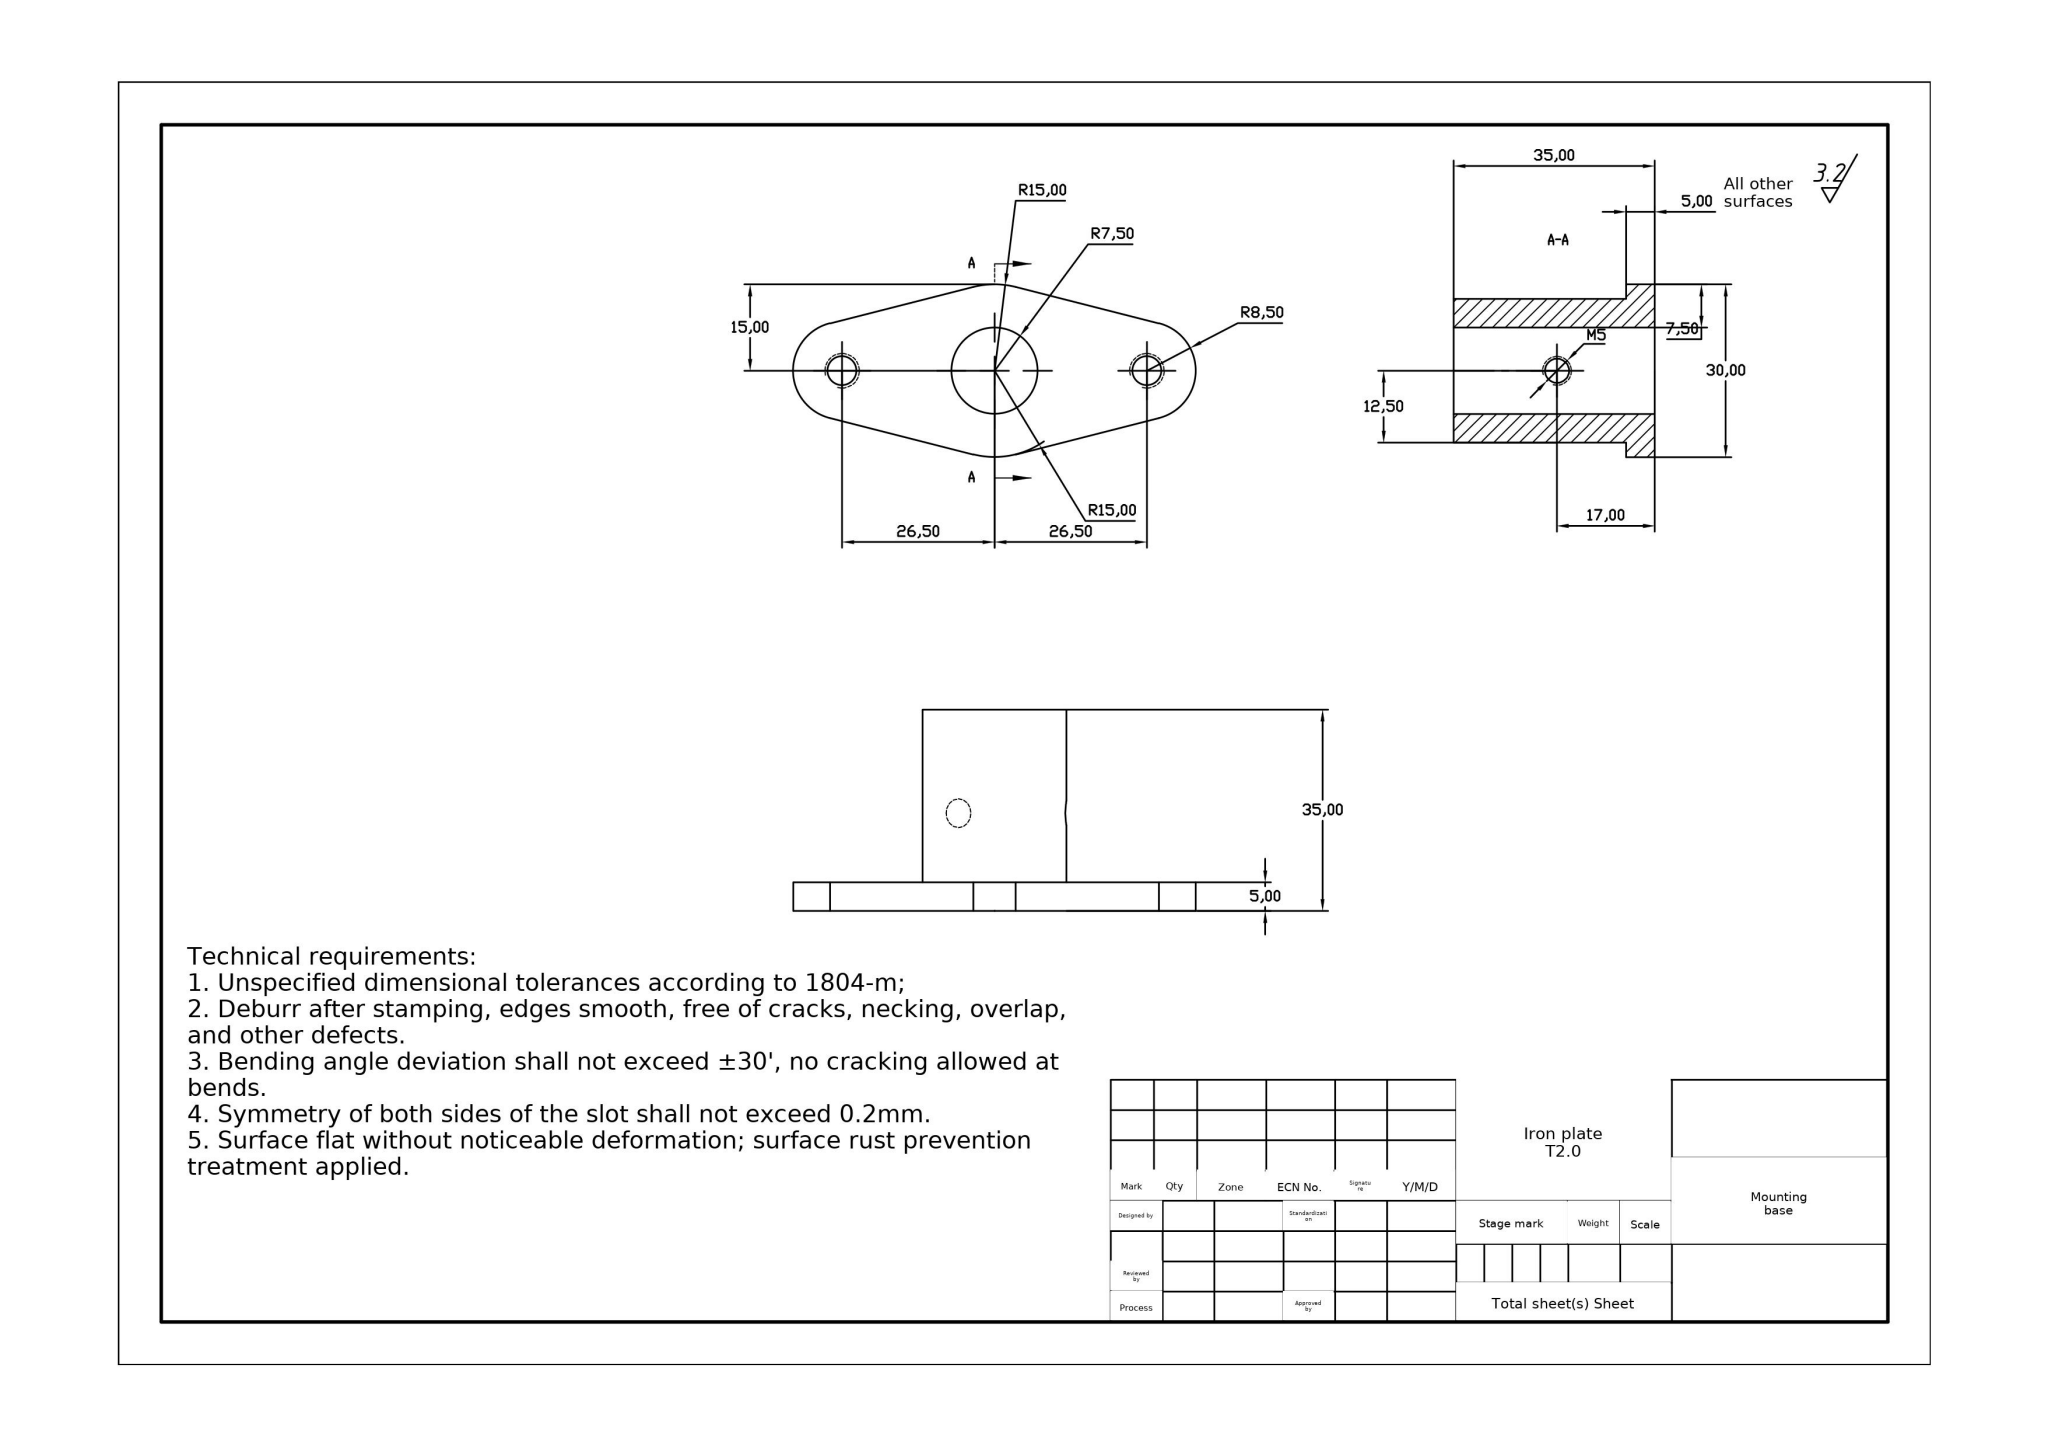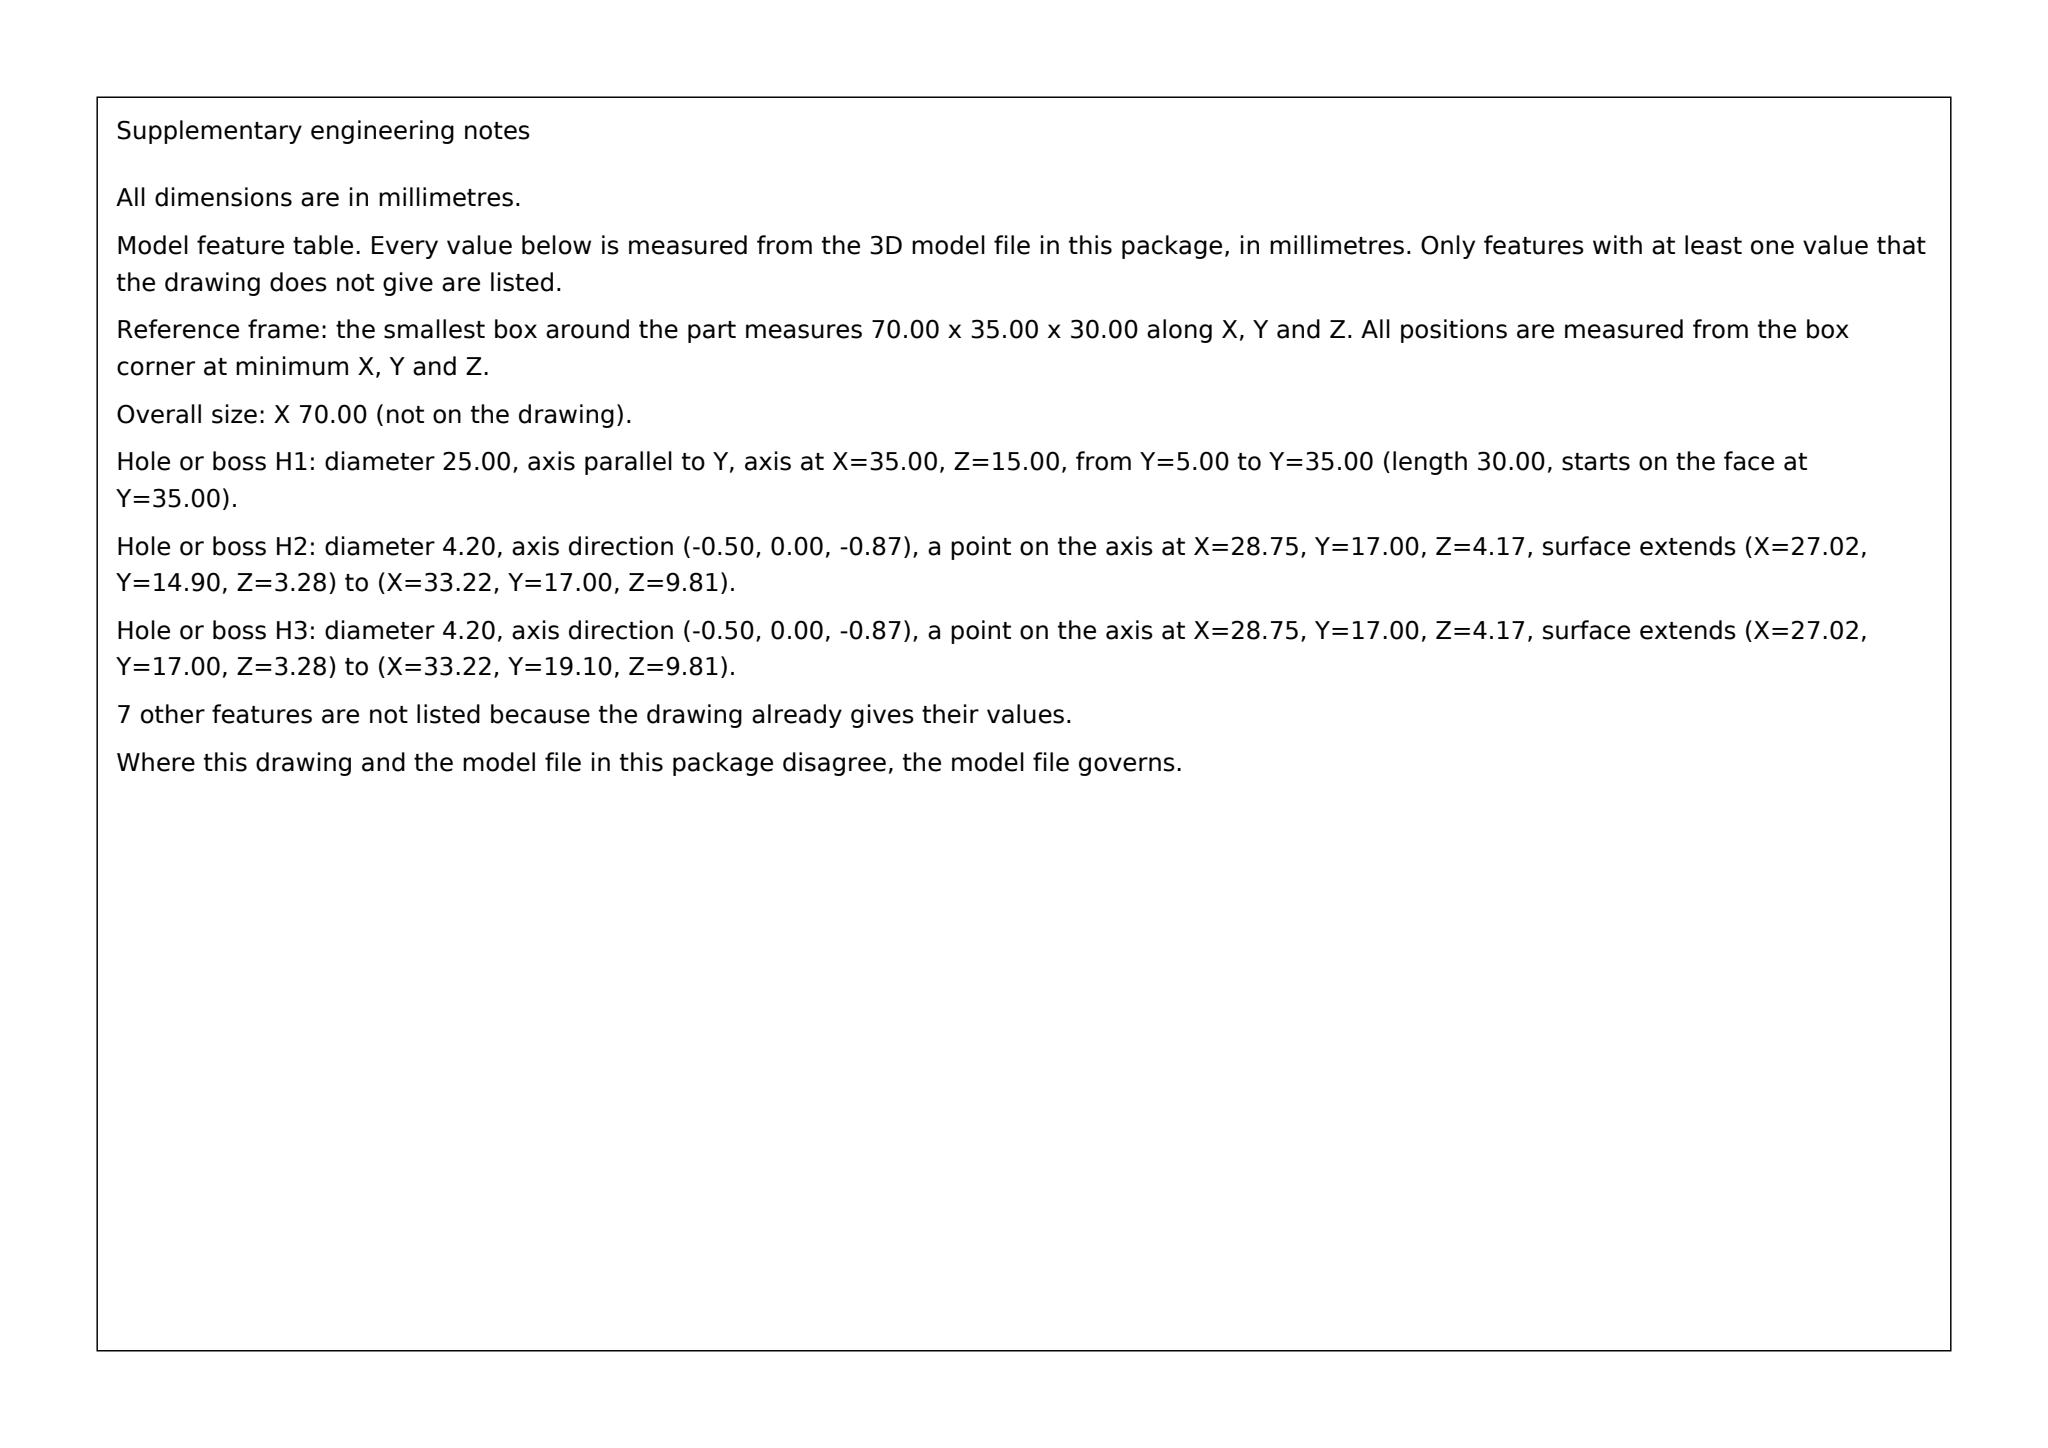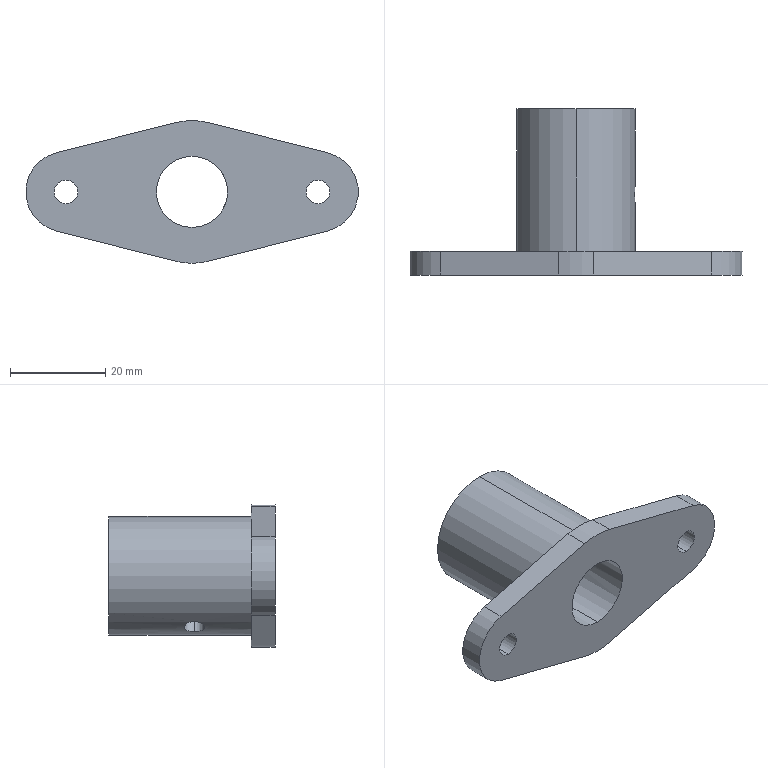Part | SolidWorks | mm | material Iron plate T2.0 | 1 solid | 24 faces | box 70 x 35 x 30 mm | volume 15756 mm3 | cylinder 17 | plane 7 | commonest cylinder face diameters 4.2 x4 5 x4 30 x3 15 x2 25 x2 17 x2
build123d program:
from build123d import *

# Parameters (mm, degrees)
BOSS_EXTRUDE1_DEPTH   = 5
M6_TAPPED_HOLE1_D     = 5
M6_TAPPED_HOLE1_DEPTH = 17
M6_TAPPED_HOLE1_TIP   = 1.502
SKETCH4_R             = 10
CUT_EXTRUDE1_DEPTH    = 10
CIRPATTERN1_COUNT     = 2
CIRPATTERN1_ANGLE     = 120


with BuildPart() as part:
    # Sketch1 → Boss-Extrude1 (new body)
    with BuildSketch(Plane(origin=(0, 0, 0), x_dir=(1, 0, 0), z_dir=(0, 1, 0))):
        with BuildLine():
            Line((-28.585, -8.24), (-3.679, -14.542))
            ThreePointArc((-3.679, -14.542), (0, -15), (3.679, -14.542))
            Line((3.679, -14.542), (28.585, -8.24))
            ThreePointArc((28.585, -8.24), (35, 0), (28.585, 8.24))
            Line((28.585, 8.24), (3.679, 14.542))
            ThreePointArc((3.679, 14.542), (0, 15), (-3.679, 14.542))
            Line((-3.679, 14.542), (-28.585, 8.24))
            ThreePointArc((-28.585, 8.24), (-35, 0), (-28.585, -8.24))
        make_face()
    extrude(amount=BOSS_EXTRUDE1_DEPTH)

    # M6 Tapped Hole1
    with Locations(Plane(origin=(-26.5, 5, 0), x_dir=(0, 0, 1), z_dir=(0, 1, 0))):
        with Locations((0, 0), (0, 53)):
            Hole(M6_TAPPED_HOLE1_D / 2, depth=M6_TAPPED_HOLE1_DEPTH)
            with Locations((0, 0, -(M6_TAPPED_HOLE1_DEPTH + M6_TAPPED_HOLE1_TIP / 2))):  # 118° drill point
                Cone(0, M6_TAPPED_HOLE1_D / 2, M6_TAPPED_HOLE1_TIP, mode=Mode.SUBTRACT)

    # Sketch4 → Cut-Extrude1 (cut)
    with BuildSketch(Plane(origin=(0, 5, 0), x_dir=(1, 0, 0), z_dir=(0, 1, 0))):
        with Locations(Location((0, 0, 0), (0, 0, 270))):
            Circle(SKETCH4_R)
    extrude(amount=-CUT_EXTRUDE1_DEPTH, mode=Mode.SUBTRACT)

    # Sketch7 → Revolve1 (revolve)
    with BuildSketch(Plane(origin=(0, 0, 0), x_dir=(0, 0, -1), z_dir=(1, 0, 0)), mode=Mode.PRIVATE) as revolve1_sk:
        Polygon((-10, 0), (-10, 5), (-12.5, 5), (-12.5, 35), (-7.5, 35), (-7.5, 0), align=None)
    revolve(revolve1_sk.sketch.rotate(Axis((0, 0, 0), (0, 1, 0)), 180), axis=Axis((0, 0, 0), (0, 1, 0)))

    # Sketch9 → M5 Tapped Hole1 (revolve, cut)
    with BuildSketch(Plane(origin=(12.5, 17, 0), x_dir=(0, 0, -1), z_dir=(0, 1, 0))):
        Polygon((0, 0), (0, 15.262), (2.1, 14), (2.1, 0), align=None)
    m5_tapped_hole1 = revolve(axis=Axis((18.85, 17, 0), (-1, 0, 0)), mode=Mode.SUBTRACT)

    # CirPattern1: M5 Tapped Hole1 ×2 about axis
    cirpattern1_axis = Axis((0, 0, 0), (0, 1, 0))
    for i in range(1, CIRPATTERN1_COUNT):
        add(m5_tapped_hole1.rotate(cirpattern1_axis, i * CIRPATTERN1_ANGLE / (CIRPATTERN1_COUNT - 1)), mode=Mode.SUBTRACT)


solid = part.part